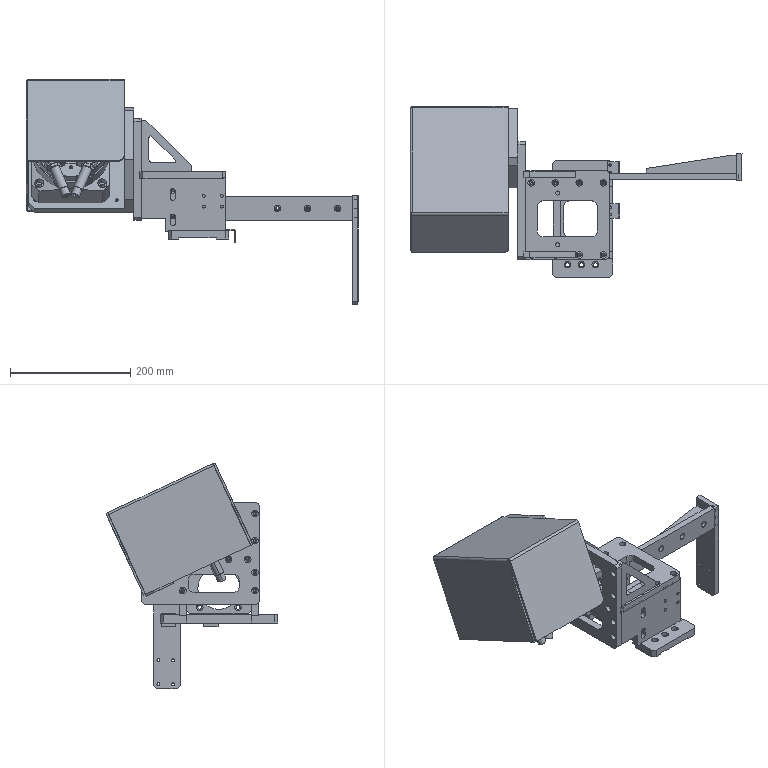Assembly | SolidWorks | mm | 26 component files | 26 solids | 1626 faces | box 552 x 284.5 x 374.42 mm | volume 3246272 mm3 | cylinder 781 | plane 565 | cone 256 | torus 20 | sphere 4 | commonest cylinder face diameters 11 x140 5 x137 6.6 x120 9 x24 15 x24 6.8 x20 8.376 x20 20 x19
Bill of materials:
17081801-804-001A | 1 | AL6061 | Thick rectangular plate with a large central rounded-rectangle through-cutout, two shallow grooves across the top face, a rectangular notch in one long edge, and a grid of round holes in mixed sizes.
17081801-804-003A | 1 | Q235 | Rectangular flange plate with chamfered corners, a large central circular through-bore, four round holes near the corners, and holes drilled into one edge face.
17081801-804-004A | 1 | AL6061 | L-shaped bracket made of two plates at a right angle. One leg has a large circular opening plus corner holes; the other leg has two arc-shaped slots and one round hole.
17081801-804-011A | 1 | Q235 | Thick, stepped rectangular plate (an L-shaped profile with one corner cut away) with two elongated slots, four small round through-holes, and a row of four holes in the top edge face.
17081801-804-012A | 1 | Q235 | Thick, stepped rectangular plate (an L-shaped profile with one corner cut away) with two elongated slots, four small round through-holes, and a row of four holes in the top edge face.
17081801-804-013A | 1 | AL6061 | Nearly square plate with chamfered corners, a large off-center rounded-rectangle through-cutout, and many round holes of mixed sizes.
17081801-804-014A | 1 | AL6061 | Rectangular plate with chamfered corners, two rounded-rectangle through-cutouts of different sizes, many round holes, and shallow grooves or a step on one face.
17081801-804-015A | 2 | AL6061 | Flat right-triangle gusset plate with a triangular through-cutout that has rounded corners.
17081801-804-017B | 2 | 1.5mm304 Stainless Steel | Thin L-shaped angle bracket with a rounded bend; one leg has two round holes.
17081801-804-022A | 1 | 3mm Cold Rolled Plate | Thin, cover-like part formed from sheet: a top panel with two downturned side flanges. On one end, the flange (or a panel) has a wide U-shaped cutout between two legs, each with a slotted hole.
17081801-804-024A | 1 | AL6061 | Long rectangular bar with through-holes in its broad face and three holes in one end face.
17081801-804-025A | 1 | AL6061 | Long, narrow rectangular plate with two chamfered corners at one end, a cluster of five round holes at the other end, and four smaller holes in a rectangular pattern.
17081801-804-026A | 1 | AL6061 | Long, narrow, wedge-shaped bar of rectangular cross-section. Its thickness increases steadily from a thin end to a thick end, and the sloped top face levels off into a short flat section at the thick end. It has three round holes in a row along one long side face and two round holes in the thick end face.
Mates:
1. coincident | 17081801-804-001A-1 face at (-18.5, 2034.4, 134) dir (0, 0, 1) | 17081801-804-017B-1 face at (22.5, 2105.9, 134) dir (0, 0, -1)
2. concentric | 17081801-804-001A-1 face at (26.5, 2123.9, 134) dir (0, 0, 1) r 1.65 | 17081801-804-017B-1 face at (26.5, 2123.9, 134) dir (0, 0, -1) r 2.25
3. concentric | 17081801-804-001A-1 face at (26.5, 2111.9, 134) dir (0, 0, 1) r 1.65 | 17081801-804-017B-1 face at (26.5, 2111.9, 134) dir (0, 0, -1) r 2.25
4. concentric | 17081801-804-001A-1 face at (-49.5, 1974.4, 120) dir (0, 0, -1) r 3.3 | 17081801-804-011A-1 face at (-49.5, 1974.4, 132) dir (0, 0, -1) r 2.5
5. concentric | 17081801-804-001A-1 face at (-29.5, 1974.4, 120) dir (0, 0, -1) r 3.3 | 17081801-804-011A-1 face at (-29.5, 1974.4, 132) dir (0, 0, -1) r 2.5
6. coincident | 17081801-804-001A-1 face at (-18.5, 2034.4, 132) dir (0, 0, 1) | 17081801-804-011A-1 face at (-54.5, 1980.4, 132) dir (0, 0, -1)
7. concentric | 17081801-804-001A-1 face at (20.5, 2094.4, 120) dir (0, 0, -1) r 3.3 | 17081801-804-012A-1 face at (20.5, 2094.4, 132) dir (0, 0, -1) r 2.5
8. concentric | 17081801-804-001A-1 face at (10.5, 2094.4, 132) dir (0, 0, 1) r 2.5 | 17081801-804-012A-1 face at (10.5, 2094.4, 132) dir (0, 0, -1) r 2.5
9. coincident | 17081801-804-001A-1 face at (-18.5, 2034.4, 132) dir (0, 0, 1) | 17081801-804-012A-1 face at (25.5, 2088.4, 132) dir (0, 0, -1)
10. width | 17081801-804-003A-1 face at (-67.9, 1980.9, 220.5) dir (0, -1, 0) | 17081801-804-003A-1 face at (-67.9, 2087.9, 220.5) dir (0, 1, 0) | 17081801-804-011A-1 face at (-54.5, 1980.4, 222) dir (0, 1, 0) | 17081801-804-012A-1 face at (25.5, 2088.4, 222) dir (0, -1, 0)
11. concentric | 17081801-804-004A-1 face at (-284, 2195.539, 286.62) dir (0, -0.9063, 0.4226) r 3.4 | 1369126_DSM_40_270_CC_HD_A_B_0-1/1369634_DSM_40_270_HD_Geh-1 face at (-284, 2195.539, 286.62) dir (0, -0.9063, 0.4226) r 4.188
12. concentric | 17081801-804-004A-1 face at (-231.5, 2186.946, 232.7) dir (0, -0.9063, 0.4226) r 63 | 1369126_DSM_40_270_CC_HD_A_B_0-1/1369634_DSM_40_270_HD_Geh-1 face at (-231.5, 2179.243, 236.292) dir (0, -0.9063, 0.4226) r 63
13. coincident | 17081801-804-004A-1 face at (-141.5, 2205.048, 307.012) dir (0, -0.9063, 0.4226) | 1369126_DSM_40_270_CC_HD_A_B_0-1/1369634_DSM_40_270_HD_Geh-1 face at (-231.5, 2173.352, 239.039) dir (0, 0.9063, -0.4226)
14. concentric | 17081801-804-004A-1 face at (-126.5, 2134.4, 191) dir (1, 0, 0) r 4.5 | 17081801-804-014A-1 face at (-126.5, 2134.4, 191) dir (-1, 0, 0) r 4.5
15. coincident | 17081801-804-004A-1 face at (-126.5, 2218.643, 300.673) dir (1, 0, 0) | 17081801-804-014A-1 face at (-126.5, 2034.4, 236) dir (-1, 0, 0)
16. angle | 17081801-804-004A-1 face at (-301.5, 2218.643, 300.673) dir (0, 0.9063, -0.4226) | 17081801-804-014A-1 face at (-120.5, 2162.4, 236) dir (0, 1, 0)
17. concentric | 17081801-804-011A-1 face at (15.5, 1974.4, 222) dir (0, 0, 1) r 2.5 | 17081801-804-013A-1 face at (15.5, 1974.4, 232) dir (0, 0, 1) r 3.3
18. coincident | 17081801-804-011A-1 face at (-54.5, 1968.4, 222) dir (0, 0, 1) | 17081801-804-013A-1 face at (-44.5, 2034.4, 222) dir (0, 0, -1)
19. concentric | 17081801-804-011A-1 face at (-24.5, 1974.4, 222) dir (0, 0, 1) r 2.5 | 17081801-804-013A-1 face at (-24.5, 1974.4, 232) dir (0, 0, 1) r 3.3
20. coincident | 17081801-804-012A-1 face at (25.5, 2100.4, 132) dir (0, 1, 0) | 17081801-804-024A-1 face at (109.25, 2100.4, 171) dir (0, -1, 0)
21. concentric | 17081801-804-012A-1 face at (19.5, 2088.4, 162) dir (0, -1, 0) r 2.5 | 17081801-804-024A-1 face at (19.5, 2110.4, 162) dir (0, 1, 0) r 3.3
22. concentric | 17081801-804-024A-1 face at (19.5, 2110.4, 180) dir (0, 1, 0) r 3.3 | 17081801-804-012A-1 face at (19.5, 2088.4, 180) dir (0, -1, 0) r 2.5
23. concentric | 17081801-804-013A-1 face at (-116.5, 2082.4, 226) dir (-1, 0, 0) r 2.5 | 17081801-804-014A-1 face at (-126.5, 2082.4, 226) dir (-1, 0, 0) r 3.3
24. concentric | 17081801-804-013A-1 face at (-116.5, 2050.4, 226) dir (-1, 0, 0) r 2.5 | 17081801-804-014A-1 face at (-126.5, 2050.4, 226) dir (-1, 0, 0) r 3.3
25. coincident | 17081801-804-013A-1 face at (-116.5, 2034.4, 226) dir (-1, 0, 0) | 17081801-804-014A-1 face at (-116.5, 2034.4, 236) dir (1, 0, 0)
26. concentric | 17081801-804-013A-1 face at (-89.5, 1974.4, 220) dir (0, 0, -1) r 3.3 | 17081801-804-015A-1 face at (-89.5, 1974.4, 232) dir (0, 0, -1) r 2.5
27. concentric | 17081801-804-013A-1 face at (-44.5, 1974.4, 220) dir (0, 0, -1) r 3.3 | 17081801-804-015A-1 face at (-44.5, 1974.4, 232) dir (0, 0, -1) r 2.5
28. coincident | 17081801-804-013A-1 face at (-44.5, 2034.4, 232) dir (0, 0, 1) | 17081801-804-015A-1 face at (-116.5, 1969.4, 232) dir (0, 0, -1)
29. concentric | 17081801-804-013A-1 face at (-89.5, 2108.4, 220) dir (0, 0, -1) r 5.5 | 17081801-804-015A-2 face at (-89.5, 2108.4, 232) dir (0, 0, -1) r 2.5
30. concentric | 17081801-804-013A-1 face at (-44.5, 2108.4, 220) dir (0, 0, -1) r 5.5 | 17081801-804-015A-2 face at (-44.5, 2108.4, 232) dir (0, 0, -1) r 2.5
31. coincident | 17081801-804-013A-1 face at (-44.5, 2034.4, 232) dir (0, 0, 1) | 17081801-804-015A-2 face at (-116.5, 2103.4, 232) dir (0, 0, -1)
32. concentric | 17081801-804-024A-1 face at (112, 2100.4, 171) dir (0, -1, 0) r 3.3 | 17081801-804-026A-1 face at (112, 2110.4, 171) dir (0, -1, 0) r 2.5
33. concentric | 17081801-804-024A-1 face at (162, 2100.4, 171) dir (0, -1, 0) r 3.3 | 17081801-804-026A-1 face at (162, 2110.4, 171) dir (0, -1, 0) r 2.5
34. coincident | 17081801-804-024A-1 face at (109.25, 2110.4, 171) dir (0, 1, 0) | 17081801-804-026A-1 face at (237, 2110.4, 166) dir (0, -1, 0)
35. concentric | 17081801-804-024A-1 face at (237, 2105.4, 186) dir (1, 0, 0) r 2.5 | 17081801-804-025A-1 face at (246, 2105.4, 186) dir (1, 0, 0) r 3.3
36. concentric | 17081801-804-024A-1 face at (237, 2105.4, 171) dir (1, 0, 0) r 2.5 | 17081801-804-025A-1 face at (246, 2105.4, 171) dir (1, 0, 0) r 5.5
37. coincident | 17081801-804-024A-1 face at (237, 2110.4, 151) dir (1, 0, 0) | 17081801-804-025A-1 face at (237, 2120.9, 101.5) dir (-1, 0, 0)
38. coincident | 17081801-804-017B-1 face at (22.5, 2105.9, 135.5) dir (0, 0, 1) | 17081801-804-017B-2 face at (22.5, 2035.9, 135.5) dir (0, 0, 1)
39. coincident | 17081801-804-017B-1 face at (42.5, 2105.9, 135.5) dir (1, 0, 0) | 17081801-804-017B-2 face at (42.5, 2035.9, 135.5) dir (1, 0, 0)
40. distance | 17081801-804-017B-2 face at (40.3, 2059.9, 133.3) dir (0, 1, 0) | 17081801-804-017B-1 face at (40.3, 2129.9, 133.3) dir (0, 1, 0)
41. distance | 17081801-804-003A-1 face at (-67.9, 2087.9, 135.5) dir (0, 0, -1) | 17081801-804-001A-1 face at (-18.5, 2034.4, 120) dir (0, 0, -1)
42. distance | 17081801-804-003A-1 face at (-67.9, 2034.4, 178) dir (-1, 0, 0) | 17081801-804-001A-1 face at (-68.5, 1936.9, 134) dir (-1, 0, 0)
43. coincident | 17081801-804-004A-1 face at (-301.5, 2218.643, 300.673) dir (0, 0.9063, -0.4226) | 17081801-804-022A-1 face at (-303, 2156.518, 167.446) dir (0, -0.9063, 0.4226)
44. width | 17081801-804-022A-1 face at (-287.75, 2153.555, 177.655) dir (-1, 0, 0) | 17081801-804-022A-1 face at (-294.25, 2153.555, 177.655) dir (1, 0, 0) | 17081801-804-004A-1 face at (-291, 2161.589, 178.321) dir (0, 0.9063, -0.4226) r 2.5
45. coincident | 17081801-804-004A-1 face at (-141.5, 2205.048, 307.012) dir (0, 0.4226, 0.9063) | 17081801-804-022A-1 face at (-303, 2221.362, 299.405) dir (0, -0.4226, -0.9063)
46. distance | 342623_DSM_40_NS-1 plane at (17.293, -30.257, 106) dir (0, 0, -1) | 1369634_DSM_40_270_HD_Geh-1 plane at (0, 0, 112) dir (0, 0, 1)
47. coincident | 1369634_DSM_40_270_HD_Geh-1 axis at (17.293, -30.257, 192.9) dir (0, 0, -1) | 342623_DSM_40_NS-1 axis at (17.293, -30.257, 17.1) dir (0, 0, 1)
48. angle | 342623_DSM_40_NS-1 plane at (17.293, -30.257, 98) dir (0.8682, 0.4962, 0) | 1369634_DSM_40_270_HD_Geh-1 plane at (0, 0, 112) dir (0.8682, 0.4962, 0)
49. distance | 704067_DSM_40_BR_HZ-1 sketch point at (17.293, -30.257, 112) dir (1, 0, 0) | 1369634_DSM_40_270_HD_Geh-1 plane at (0, 0, 112) dir (0, 0, 1)
50. coincident | 1369634_DSM_40_270_HD_Geh-1 axis at (17.293, -30.257, 192.9) dir (0, 0, -1) | 704067_DSM_40_BR_HZ-1 sketch point at (17.293, -30.257, 112) dir (1, 0, 0)
51. angle | 1369634_DSM_40_270_HD_Geh-1 axis at (-17.25, -50, 112) dir (0.8682, 0.4962, 0) | 704067_DSM_40_BR_HZ-1 axis at (-57.9, -0.4098, 112) dir (0.9295, -0.3689, 0)
52. angle | 1369634_DSM_40_270_HD_Geh-1 axis at (17.293, -30.257, 192.9) dir (0, 0, -1) | 704067_DSM_40_BR_HZ-1 axis at (17.293, -30.257, 216.9) dir (0, 0, -1)
53. distance | 548014_DYSC_12_12_Y1F_SD_0-1 sketch point at (37.468, -26.865, 124.7) dir (1, 0, 0) | 704067_DSM_40_BR_HZ-1 plane at (20.206, -22.918, 136) dir (0.3689, 0.9295, 0)
54. coincident | 704067_DSM_40_BR_HZ-1 axis at (52.005, 9.76, 124.7) dir (-0.3689, -0.9295, 0) | 548014_DYSC_12_12_Y1F_SD_0-1 sketch point at (37.468, -26.865, 124.7) dir (1, 0, 0)
55. angle | 704067_DSM_40_BR_HZ-1 axis at (-54.987, 6.929, 124.7) dir (0.9295, -0.3689, 0) | 548014_DYSC_12_12_Y1F_SD_0-1 axis at (-37.725, 2.982, 124.7) dir (0.9295, -0.3689, 0)
56. angle | 704067_DSM_40_BR_HZ-1 axis at (52.005, 9.76, 124.7) dir (-0.3689, -0.9295, 0) | 548014_DYSC_12_12_Y1F_SD_0-1 axis at (67.315, 48.328, 124.7) dir (-0.3689, -0.9295, 0)
57. distance | Flachmutter_M16x1_5_20-1 plane at (28.724, -48.893, 124.7) dir (-0.3689, -0.9295, 0) | 704067_DSM_40_BR_HZ-1 plane at (12.459, -42.436, 136) dir (0.3689, 0.9295, 0)
58. coincident | 704067_DSM_40_BR_HZ-1 axis at (52.005, 9.76, 124.7) dir (-0.3689, -0.9295, 0) | Flachmutter_M16x1_5_20-1 axis at (-1.123, -124.086, 124.7) dir (0.3689, 0.9295, 0)
59. angle | Flachmutter_M16x1_5_20-1 plane at (28.724, -48.893, 124.7) dir (0.8049, -0.3195, -0.5) | 704067_DSM_40_BR_HZ-1 plane at (33.559, -36.713, 136) dir (0.9295, -0.3689, 0)
60. distance | 342623_DSM_40_NS-2 plane at (-17.293, -30.257, 106) dir (0, 0, -1) | 1369634_DSM_40_270_HD_Geh-1 plane at (0, 0, 112) dir (0, 0, 1)
61. coincident | 1369634_DSM_40_270_HD_Geh-1 axis at (-17.293, -30.257, 192.9) dir (0, 0, -1) | 342623_DSM_40_NS-2 axis at (-17.293, -30.257, 17.1) dir (0, 0, 1)
62. angle | 342623_DSM_40_NS-2 plane at (-17.293, -30.257, 98) dir (0.8682, -0.4962, 0) | 1369634_DSM_40_270_HD_Geh-1 plane at (0, 0, 112) dir (0.8682, -0.4962, 0)
63. distance | 704066_DSM_40_BL_HZ-1 sketch point at (-17.293, -30.257, 112) dir (1, 0, 0) | 1369634_DSM_40_270_HD_Geh-1 plane at (0, 0, 112) dir (0, 0, 1)
64. coincident | 1369634_DSM_40_270_HD_Geh-1 axis at (-17.293, -30.257, 192.9) dir (0, 0, -1) | 704066_DSM_40_BL_HZ-1 sketch point at (-17.293, -30.257, 112) dir (1, 0, 0)
65. angle | 1369634_DSM_40_270_HD_Geh-1 axis at (-80.9, 6.098, 112) dir (0.8682, -0.4962, 0) | 704066_DSM_40_BL_HZ-1 axis at (57.9, -0.4098, 112) dir (-0.9295, -0.3689, 0)
66. angle | 1369634_DSM_40_270_HD_Geh-1 axis at (-17.293, -30.257, 192.9) dir (0, 0, -1) | 704066_DSM_40_BL_HZ-1 axis at (-17.293, -30.257, 216.9) dir (0, 0, -1)
67. distance | 548014_DYSC_12_12_Y1F_SD_0-2 plane at (-37.468, -26.865, 124.7) dir (-0.3689, 0.9295, 0) | 704066_DSM_40_BL_HZ-1 plane at (-20.206, -22.918, 136) dir (0.3689, -0.9295, 0)
68. coincident | 704066_DSM_40_BL_HZ-1 axis at (-15.112, -83.186, 124.7) dir (-0.3689, 0.9295, 0) | 548014_DYSC_12_12_Y1F_SD_0-2 axis at (-67.315, 48.328, 124.7) dir (0.3689, -0.9295, 0)
69. angle | 548014_DYSC_12_12_Y1F_SD_0-2 plane at (-37.468, -26.865, 124.7) dir (-0.9295, -0.3689, 0) | 704066_DSM_40_BL_HZ-1 plane at (-33.559, -36.713, 136) dir (-0.9295, -0.3689, 0)
70. coincident | 704066_DSM_40_BL_HZ-1 axis at (-17.293, -30.257, 216.9) dir (0, 0, -1) | DIN_912_M8x30_F-2 sketch point at (-17.293, -30.257, 128) dir (1, 0, 0)
71. angle | 704066_DSM_40_BL_HZ-1 axis at (57.9, -0.4098, 127.4) dir (-0.9295, -0.3689, 0) | DIN_912_M8x30_F-2 axis at (57.9, -0.4098, 128) dir (-0.9295, -0.3689, 0)
72. angle | 704066_DSM_40_BL_HZ-1 axis at (-17.293, -30.257, 216.9) dir (0, 0, -1) | DIN_912_M8x30_F-2 axis at (-17.293, -30.257, 178) dir (0, 0, -1)
73. distance | Flachmutter_M16x1_5_20-2 plane at (-28.724, -48.893, 124.7) dir (0.3689, -0.9295, 0) | 704066_DSM_40_BL_HZ-1 plane at (-12.459, -42.436, 136) dir (-0.3689, 0.9295, 0)
74. coincident | 704066_DSM_40_BL_HZ-1 axis at (-52.005, 9.76, 124.7) dir (0.3689, -0.9295, 0) | Flachmutter_M16x1_5_20-2 axis at (1.123, -124.086, 124.7) dir (-0.3689, 0.9295, 0)
75. angle | Flachmutter_M16x1_5_20-2 plane at (-28.724, -48.893, 124.7) dir (-0.8049, -0.3195, 0.5) | 704066_DSM_40_BL_HZ-1 plane at (-33.559, -36.713, 136) dir (-0.9295, -0.3689, 0)
76. coincident | 1369634_DSM_40_270_HD_Geh-1 plane at (0, 0, 0) dir (0, 0, -1) | 1369634_DSM_40_270_HD_Kol-1 plane at (0, 0, 0) dir (0, 0, 1)
77. coincident | 1369634_DSM_40_270_HD_Geh-1 axis at (0, 0, 31.1) dir (0, 0, 1) | 1369634_DSM_40_270_HD_Kol-1 axis at (0, 0, 234.9) dir (0, 0, -1)